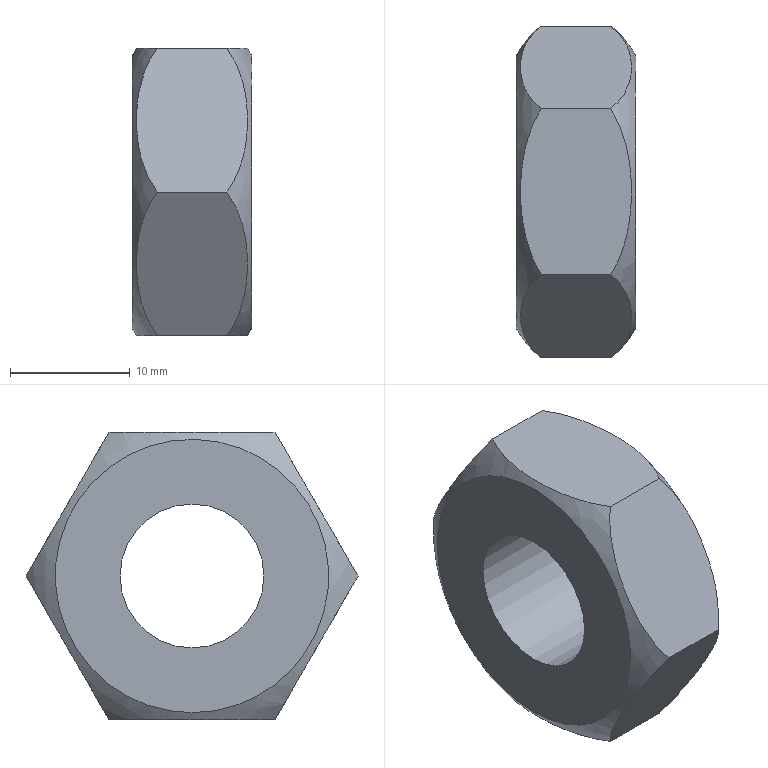Component | NX | NUT_M12_2 | 1 solid | 11 faces | volume 3768 mm3 | plane 8 | spline 2 | cylinder 1 | commonest cylinder face diameters 12 x1